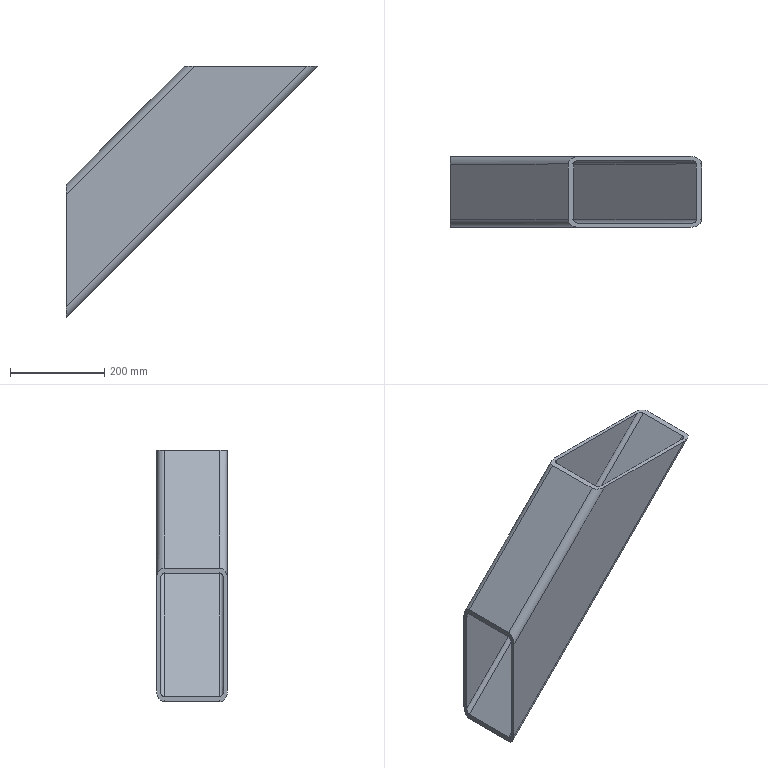Component | NX | AAAAAAAAAAAAAAAAAAAAAAAAAAAAAAAAAAAAAAAAAAAAAAAAAAAAAAAAAAA | 1 solid | 18 faces | volume 2866956 mm3 | plane 10 | cylinder 8 | commonest cylinder face diameters 32 x4 16 x4